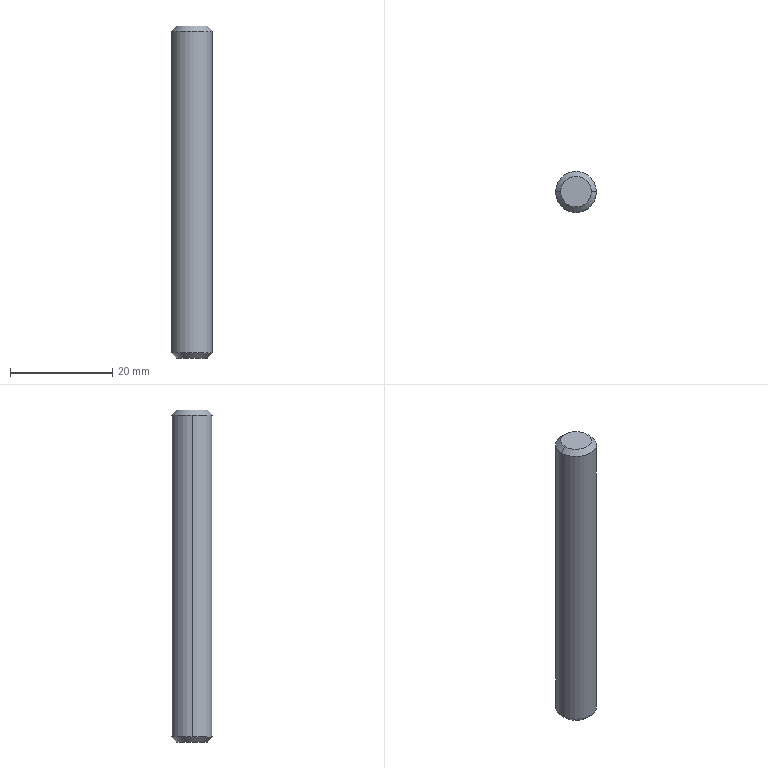Component | SolidWorks | AdjustingBoltAssembly9.26-1_UpperBaffleAdjustmentBolt9.26-1 | 1 solid | 8 faces | box 8 x 8 x 65 mm | volume 3244 mm3 | cone 4 | cylinder 2 | plane 2 | commonest cylinder face diameters 8 x2
build123d program:
from build123d import *

# Parameters (mm, degrees)
SKETCH1_R           = 4
BOSS_EXTRUDE1_DEPTH = 65
CHAMFER1_SIZE       = 1


with BuildPart() as part:
    # Sketch1 → Boss-Extrude1 (new body)
    with BuildSketch(Plane.XY):
        Circle(SKETCH1_R)
    extrude(amount=BOSS_EXTRUDE1_DEPTH)

    # Chamfer1
    chamfer1_edges = [part.edges().sort_by_distance(p)[0] for p in [
        (-4, 0, 0),
        (-4, 0, 65),
    ]]
    chamfer(chamfer1_edges, length=CHAMFER1_SIZE)


solid = part.part

# Placed as in the assembly
solid = solid.moved(Location((100, 52.697, -17.25), (0, 0, 0)))